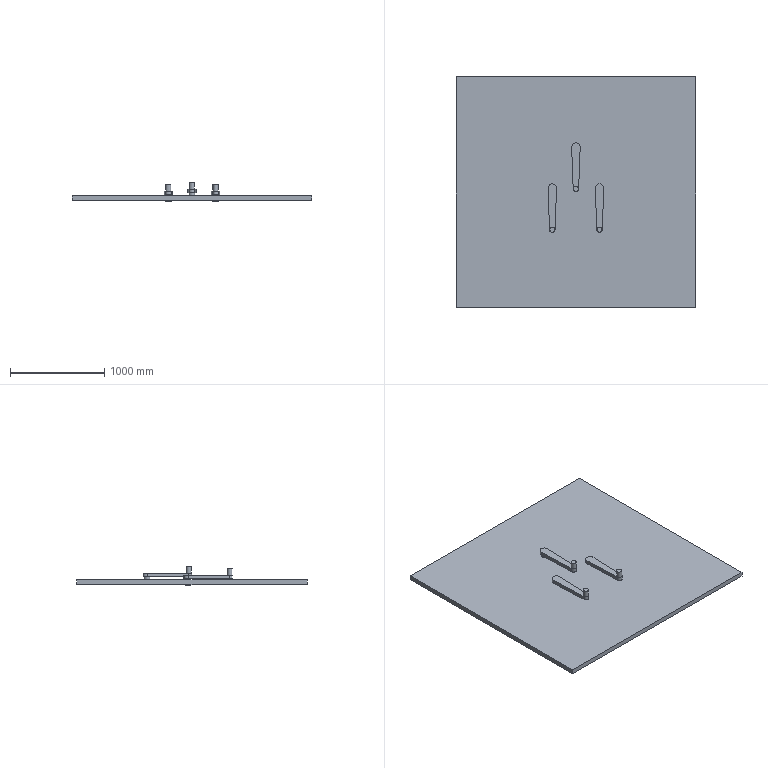Assembly | NX | mm | 4 component files | 4 solids | 39 faces | box 2530 x 2440 x 200 mm | volume 313761374 mm3 | plane 24 | cylinder 15 | commonest cylinder face diameters 60 x6 58 x3 90 x3 54 x3
Bill of materials:
unnamed part 1 | 1 |  | Flat, tapered arm with rounded ends. A solid cylindrical boss sticks up from the narrow end, and a slightly larger cylindrical boss sticks down from the wide end, on the opposite face.
unnamed part 2 | 1 |  | Flat, tapered arm with rounded ends. A solid cylindrical boss sticks up from the narrow end, and a slightly larger cylindrical boss sticks down from the wide end, on the opposite face.
unnamed part 3 | 1 |  | Thin, flat plate, square or nearly square, with three small round through-holes near the center arranged in a triangle.
unnamed part 4 | 1 |  | Flat, tapered arm with rounded ends. A solid cylindrical boss sticks up from the narrow end, and a slightly larger cylindrical boss sticks down from the wide end, on the opposite face.
Mates:
1. touch align | part_2 1 face | assembly face
2. concentric | part_2 1 nxobject | part_3 1 edge
3. concentric | part_2 1 nxobject | part_4 1 edge